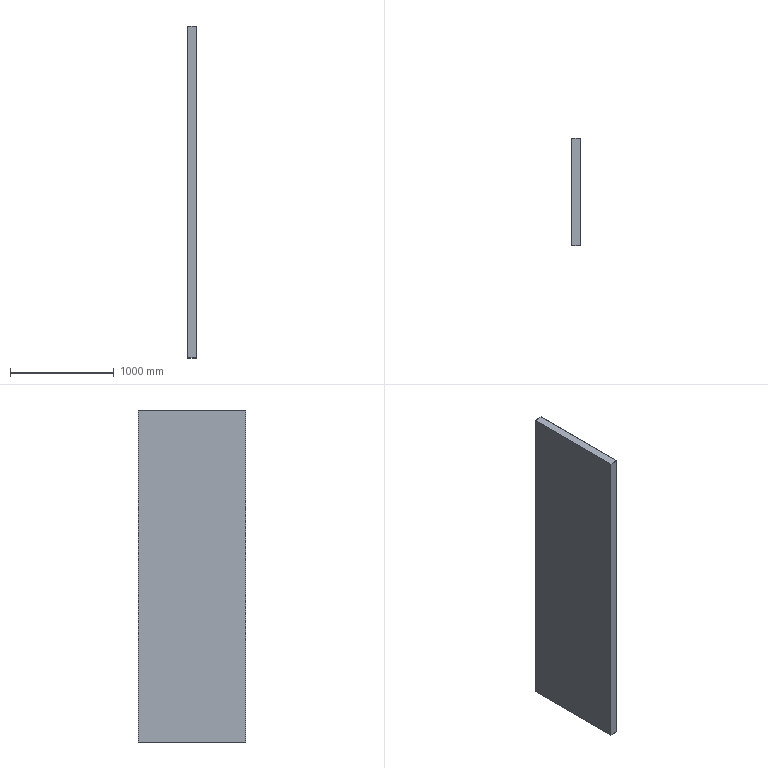Component | NX | DS1 | 1 solid | 15 faces | volume 6080082 mm3 | plane 15